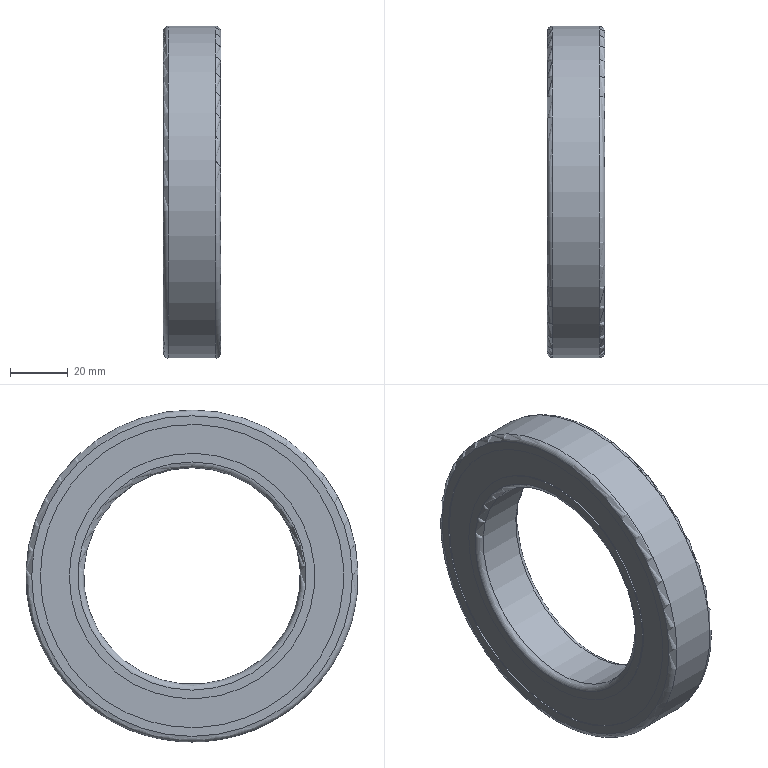Component | NX | BEARING_1 | 1 solid | 16 faces | box 20 x 115 x 115 mm | volume 115371 mm3 | plane 6 | cylinder 6 | torus 4 | commonest cylinder face diameters 105 x2 85 x2 115 x1 75 x1
STEP:
#1=CARTESIAN_POINT('',(0.,0.,0.));
#2=DIRECTION('',(0.,0.,1.));
#3=DIRECTION('',(1.,0.,0.));
#4=AXIS2_PLACEMENT_3D('',#1,#2,#3);
#5=CARTESIAN_POINT('',(1318.754,222.349,517.977));
#6=VERTEX_POINT('',#5);
#7=CARTESIAN_POINT('',(1318.754,222.349,478.477));
#8=DIRECTION('',(1.,0.,0.));
#9=DIRECTION('',(0.,0.,1.));
#10=AXIS2_PLACEMENT_3D('',#7,#8,#9);
#11=CIRCLE('',#10,39.5);
#12=CARTESIAN_POINT('',(1318.754,222.349,478.477));
#13=DIRECTION('',(1.,0.,0.));
#14=DIRECTION('',(0.,0.,1.));
#15=AXIS2_PLACEMENT_3D('',#12,#13,#14);
#16=PLANE('',#15);
#17=CARTESIAN_POINT('',(0.,0.));
#18=DIRECTION('',(1.,0.));
#19=AXIS2_PLACEMENT_2D('',#17,#18);
#20=CIRCLE('',#19,39.5);
#21=(GEOMETRIC_REPRESENTATION_CONTEXT(2)PARAMETRIC_REPRESENTATION_CONTEXT()REPRESENTATION_CONTEXT('',''));
#22=DEFINITIONAL_REPRESENTATION('',(#20),#21);
#23=PCURVE('',#16,#22);
#24=CARTESIAN_POINT('',(1320.754,222.349,478.477));
#25=DIRECTION('',(1.,0.,0.));
#26=DIRECTION('',(0.,0.,1.));
#27=AXIS2_PLACEMENT_3D('',#24,#25,#26);
#28=TOROIDAL_SURFACE('',#27,39.5,2.);
#29=CARTESIAN_POINT('',(0.,4.712));
#30=DIRECTION('',(1.,0.));
#31=VECTOR('',#30,1.);
#32=LINE('',#29,#31);
#33=(GEOMETRIC_REPRESENTATION_CONTEXT(2)PARAMETRIC_REPRESENTATION_CONTEXT()REPRESENTATION_CONTEXT('',''));
#34=DEFINITIONAL_REPRESENTATION('',(#32),#33);
#35=PCURVE('',#28,#34);
#36=SURFACE_CURVE('',#11,(#23,#35),.PCURVE_S1.);
#37=EDGE_CURVE('',#6,#6,#36,.T.);
#38=ORIENTED_EDGE('',*,*,#37,.T.);
#39=EDGE_LOOP('',(#38));
#40=FACE_BOUND('',#39,.T.);
#41=CARTESIAN_POINT('',(1318.754,264.849,478.477));
#42=VERTEX_POINT('',#41);
#43=CARTESIAN_POINT('',(1318.754,222.349,478.477));
#44=DIRECTION('',(-1.,0.,0.));
#45=DIRECTION('',(0.,1.,0.));
#46=AXIS2_PLACEMENT_3D('',#43,#44,#45);
#47=CIRCLE('',#46,42.5);
#48=CARTESIAN_POINT('',(0.,-42.5));
#49=CARTESIAN_POINT('',(-73.612,-42.5));
#50=CARTESIAN_POINT('',(-36.806,21.25));
#51=CARTESIAN_POINT('',(-0.,85.));
#52=CARTESIAN_POINT('',(36.806,21.25));
#53=CARTESIAN_POINT('',(73.612,-42.5));
#54=CARTESIAN_POINT('',(0.,-42.5));
#55=(BOUNDED_CURVE()B_SPLINE_CURVE(2,(#48,#49,#50,#51,#52,#53,#54),.UNSPECIFIED.,.T.,.F.)B_SPLINE_CURVE_WITH_KNOTS((1,2,2,2,2,1),(-2.094,0.,2.094,4.189,6.283,8.378),.UNSPECIFIED.)CURVE()GEOMETRIC_REPRESENTATION_ITEM()RATIONAL_B_SPLINE_CURVE((1.,0.5,1.,0.5,1.,0.5,1.))REPRESENTATION_ITEM(''));
#56=(GEOMETRIC_REPRESENTATION_CONTEXT(2)PARAMETRIC_REPRESENTATION_CONTEXT()REPRESENTATION_CONTEXT('',''));
#57=DEFINITIONAL_REPRESENTATION('',(#55),#56);
#58=PCURVE('',#16,#57);
#59=CARTESIAN_POINT('',(1319.254,222.349,478.477));
#60=DIRECTION('',(-1.,0.,0.));
#61=DIRECTION('',(0.,0.,-1.));
#62=AXIS2_PLACEMENT_3D('',#59,#60,#61);
#63=CYLINDRICAL_SURFACE('',#62,42.5);
#64=CARTESIAN_POINT('',(4.712,0.5));
#65=DIRECTION('',(1.,0.));
#66=VECTOR('',#65,1.);
#67=LINE('',#64,#66);
#68=(GEOMETRIC_REPRESENTATION_CONTEXT(2)PARAMETRIC_REPRESENTATION_CONTEXT()REPRESENTATION_CONTEXT('',''));
#69=DEFINITIONAL_REPRESENTATION('',(#67),#68);
#70=PCURVE('',#63,#69);
#71=SURFACE_CURVE('',#47,(#58,#70),.PCURVE_S1.);
#72=EDGE_CURVE('',#42,#42,#71,.T.);
#73=ORIENTED_EDGE('',*,*,#72,.T.);
#74=EDGE_LOOP('',(#73));
#75=FACE_BOUND('',#74,.T.);
#76=ADVANCED_FACE('',(#40,#75),#16,.F.);
#77=CARTESIAN_POINT('',(1320.754,222.349,535.977));
#78=VERTEX_POINT('',#77);
#79=CARTESIAN_POINT('',(1320.754,222.349,478.477));
#80=DIRECTION('',(1.,0.,0.));
#81=DIRECTION('',(0.,0.,1.));
#82=AXIS2_PLACEMENT_3D('',#79,#80,#81);
#83=CIRCLE('',#82,57.5);
#84=CARTESIAN_POINT('',(1328.754,222.349,478.477));
#85=DIRECTION('',(-1.,0.,0.));
#86=DIRECTION('',(0.,0.,-1.));
#87=AXIS2_PLACEMENT_3D('',#84,#85,#86);
#88=CYLINDRICAL_SURFACE('',#87,57.5);
#89=CARTESIAN_POINT('',(9.425,8.));
#90=DIRECTION('',(-1.,0.));
#91=VECTOR('',#90,1.);
#92=LINE('',#89,#91);
#93=(GEOMETRIC_REPRESENTATION_CONTEXT(2)PARAMETRIC_REPRESENTATION_CONTEXT()REPRESENTATION_CONTEXT('',''));
#94=DEFINITIONAL_REPRESENTATION('',(#92),#93);
#95=PCURVE('',#88,#94);
#96=CARTESIAN_POINT('',(1320.754,222.349,478.477));
#97=DIRECTION('',(1.,0.,0.));
#98=DIRECTION('',(0.,0.,1.));
#99=AXIS2_PLACEMENT_3D('',#96,#97,#98);
#100=TOROIDAL_SURFACE('',#99,55.5,2.);
#101=CARTESIAN_POINT('',(0.,6.283));
#102=DIRECTION('',(1.,0.));
#103=VECTOR('',#102,1.);
#104=LINE('',#101,#103);
#105=(GEOMETRIC_REPRESENTATION_CONTEXT(2)PARAMETRIC_REPRESENTATION_CONTEXT()REPRESENTATION_CONTEXT('',''));
#106=DEFINITIONAL_REPRESENTATION('',(#104),#105);
#107=PCURVE('',#100,#106);
#108=SURFACE_CURVE('',#83,(#95,#107),.PCURVE_S1.);
#109=EDGE_CURVE('',#78,#78,#108,.T.);
#110=ORIENTED_EDGE('',*,*,#109,.T.);
#111=CARTESIAN_POINT('',(1336.754,222.349,535.977));
#112=VERTEX_POINT('',#111);
#113=CARTESIAN_POINT('',(1336.754,222.349,535.977));
#114=CARTESIAN_POINT('',(1320.754,222.349,535.977));
#115=B_SPLINE_CURVE_WITH_KNOTS('',1,(#113,#114),.UNSPECIFIED.,.F.,.F.,(2,2),(-8.,8.),.PIECEWISE_BEZIER_KNOTS.);
#116=CARTESIAN_POINT('',(3.142,0.));
#117=DIRECTION('',(0.,1.));
#118=VECTOR('',#117,1.);
#119=LINE('',#116,#118);
#120=(GEOMETRIC_REPRESENTATION_CONTEXT(2)PARAMETRIC_REPRESENTATION_CONTEXT()REPRESENTATION_CONTEXT('',''));
#121=DEFINITIONAL_REPRESENTATION('',(#119),#120);
#122=PCURVE('',#88,#121);
#123=CARTESIAN_POINT('',(9.425,0.));
#124=DIRECTION('',(0.,1.));
#125=VECTOR('',#124,1.);
#126=LINE('',#123,#125);
#127=(GEOMETRIC_REPRESENTATION_CONTEXT(2)PARAMETRIC_REPRESENTATION_CONTEXT()REPRESENTATION_CONTEXT('',''));
#128=DEFINITIONAL_REPRESENTATION('',(#126),#127);
#129=PCURVE('',#88,#128);
#130=SEAM_CURVE('',#115,(#122,#129),.PCURVE_S1.);
#131=EDGE_CURVE('',#112,#78,#130,.T.);
#132=ORIENTED_EDGE('',*,*,#131,.F.);
#133=CARTESIAN_POINT('',(1336.754,222.349,478.477));
#134=DIRECTION('',(-1.,0.,0.));
#135=DIRECTION('',(0.,0.,1.));
#136=AXIS2_PLACEMENT_3D('',#133,#134,#135);
#137=CIRCLE('',#136,57.5);
#138=CARTESIAN_POINT('',(3.142,-8.));
#139=DIRECTION('',(1.,0.));
#140=VECTOR('',#139,1.);
#141=LINE('',#138,#140);
#142=(GEOMETRIC_REPRESENTATION_CONTEXT(2)PARAMETRIC_REPRESENTATION_CONTEXT()REPRESENTATION_CONTEXT('',''));
#143=DEFINITIONAL_REPRESENTATION('',(#141),#142);
#144=PCURVE('',#88,#143);
#145=CARTESIAN_POINT('',(1336.754,222.349,478.477));
#146=DIRECTION('',(-1.,0.,0.));
#147=DIRECTION('',(0.,0.,1.));
#148=AXIS2_PLACEMENT_3D('',#145,#146,#147);
#149=TOROIDAL_SURFACE('',#148,55.5,2.);
#150=CARTESIAN_POINT('',(0.,6.283));
#151=DIRECTION('',(1.,0.));
#152=VECTOR('',#151,1.);
#153=LINE('',#150,#152);
#154=(GEOMETRIC_REPRESENTATION_CONTEXT(2)PARAMETRIC_REPRESENTATION_CONTEXT()REPRESENTATION_CONTEXT('',''));
#155=DEFINITIONAL_REPRESENTATION('',(#153),#154);
#156=PCURVE('',#149,#155);
#157=SURFACE_CURVE('',#137,(#144,#156),.PCURVE_S1.);
#158=EDGE_CURVE('',#112,#112,#157,.T.);
#159=ORIENTED_EDGE('',*,*,#158,.T.);
#160=ORIENTED_EDGE('',*,*,#131,.T.);
#161=EDGE_LOOP('',(#110,#132,#159,#160));
#162=FACE_BOUND('',#161,.T.);
#163=ADVANCED_FACE('',(#162),#88,.T.);
#164=CARTESIAN_POINT('',(1320.754,222.349,515.977));
#165=VERTEX_POINT('',#164);
#166=CARTESIAN_POINT('',(1320.754,222.349,478.477));
#167=DIRECTION('',(-1.,0.,0.));
#168=DIRECTION('',(0.,0.,1.));
#169=AXIS2_PLACEMENT_3D('',#166,#167,#168);
#170=CIRCLE('',#169,37.5);
#171=CARTESIAN_POINT('',(1328.754,222.349,478.477));
#172=DIRECTION('',(-1.,0.,0.));
#173=DIRECTION('',(0.,0.,-1.));
#174=AXIS2_PLACEMENT_3D('',#171,#172,#173);
#175=CYLINDRICAL_SURFACE('',#174,37.5);
#176=CARTESIAN_POINT('',(3.142,8.));
#177=DIRECTION('',(1.,0.));
#178=VECTOR('',#177,1.);
#179=LINE('',#176,#178);
#180=(GEOMETRIC_REPRESENTATION_CONTEXT(2)PARAMETRIC_REPRESENTATION_CONTEXT()REPRESENTATION_CONTEXT('',''));
#181=DEFINITIONAL_REPRESENTATION('',(#179),#180);
#182=PCURVE('',#175,#181);
#183=CARTESIAN_POINT('',(6.283,3.142));
#184=DIRECTION('',(-1.,0.));
#185=VECTOR('',#184,1.);
#186=LINE('',#183,#185);
#187=(GEOMETRIC_REPRESENTATION_CONTEXT(2)PARAMETRIC_REPRESENTATION_CONTEXT()REPRESENTATION_CONTEXT('',''));
#188=DEFINITIONAL_REPRESENTATION('',(#186),#187);
#189=PCURVE('',#28,#188);
#190=SURFACE_CURVE('',#170,(#182,#189),.PCURVE_S1.);
#191=EDGE_CURVE('',#165,#165,#190,.T.);
#192=ORIENTED_EDGE('',*,*,#191,.F.);
#193=CARTESIAN_POINT('',(1336.754,222.349,515.977));
#194=VERTEX_POINT('',#193);
#195=CARTESIAN_POINT('',(1336.754,222.349,515.977));
#196=CARTESIAN_POINT('',(1320.754,222.349,515.977));
#197=B_SPLINE_CURVE_WITH_KNOTS('',1,(#195,#196),.UNSPECIFIED.,.F.,.F.,(2,2),(-8.,8.),.PIECEWISE_BEZIER_KNOTS.);
#198=CARTESIAN_POINT('',(3.142,0.));
#199=DIRECTION('',(0.,1.));
#200=VECTOR('',#199,1.);
#201=LINE('',#198,#200);
#202=(GEOMETRIC_REPRESENTATION_CONTEXT(2)PARAMETRIC_REPRESENTATION_CONTEXT()REPRESENTATION_CONTEXT('',''));
#203=DEFINITIONAL_REPRESENTATION('',(#201),#202);
#204=PCURVE('',#175,#203);
#205=CARTESIAN_POINT('',(9.425,0.));
#206=DIRECTION('',(0.,1.));
#207=VECTOR('',#206,1.);
#208=LINE('',#205,#207);
#209=(GEOMETRIC_REPRESENTATION_CONTEXT(2)PARAMETRIC_REPRESENTATION_CONTEXT()REPRESENTATION_CONTEXT('',''));
#210=DEFINITIONAL_REPRESENTATION('',(#208),#209);
#211=PCURVE('',#175,#210);
#212=SEAM_CURVE('',#197,(#204,#211),.PCURVE_S1.);
#213=EDGE_CURVE('',#194,#165,#212,.T.);
#214=ORIENTED_EDGE('',*,*,#213,.F.);
#215=CARTESIAN_POINT('',(1336.754,222.349,478.477));
#216=DIRECTION('',(1.,0.,0.));
#217=DIRECTION('',(0.,0.,1.));
#218=AXIS2_PLACEMENT_3D('',#215,#216,#217);
#219=CIRCLE('',#218,37.5);
#220=CARTESIAN_POINT('',(9.425,-8.));
#221=DIRECTION('',(-1.,0.));
#222=VECTOR('',#221,1.);
#223=LINE('',#220,#222);
#224=(GEOMETRIC_REPRESENTATION_CONTEXT(2)PARAMETRIC_REPRESENTATION_CONTEXT()REPRESENTATION_CONTEXT('',''));
#225=DEFINITIONAL_REPRESENTATION('',(#223),#224);
#226=PCURVE('',#175,#225);
#227=CARTESIAN_POINT('',(1336.754,222.349,478.477));
#228=DIRECTION('',(-1.,0.,0.));
#229=DIRECTION('',(0.,0.,1.));
#230=AXIS2_PLACEMENT_3D('',#227,#228,#229);
#231=TOROIDAL_SURFACE('',#230,39.5,2.);
#232=CARTESIAN_POINT('',(6.283,3.142));
#233=DIRECTION('',(-1.,0.));
#234=VECTOR('',#233,1.);
#235=LINE('',#232,#234);
#236=(GEOMETRIC_REPRESENTATION_CONTEXT(2)PARAMETRIC_REPRESENTATION_CONTEXT()REPRESENTATION_CONTEXT('',''));
#237=DEFINITIONAL_REPRESENTATION('',(#235),#236);
#238=PCURVE('',#231,#237);
#239=SURFACE_CURVE('',#219,(#226,#238),.PCURVE_S1.);
#240=EDGE_CURVE('',#194,#194,#239,.T.);
#241=ORIENTED_EDGE('',*,*,#240,.F.);
#242=ORIENTED_EDGE('',*,*,#213,.T.);
#243=EDGE_LOOP('',(#192,#214,#241,#242));
#244=FACE_BOUND('',#243,.F.);
#245=ADVANCED_FACE('',(#244),#175,.F.);
#246=CARTESIAN_POINT('',(1318.754,222.349,533.977));
#247=VERTEX_POINT('',#246);
#248=CARTESIAN_POINT('',(1318.754,222.349,478.477));
#249=DIRECTION('',(-1.,0.,0.));
#250=DIRECTION('',(0.,0.,1.));
#251=AXIS2_PLACEMENT_3D('',#248,#249,#250);
#252=CIRCLE('',#251,55.5);
#253=CARTESIAN_POINT('',(1318.754,222.349,478.477));
#254=DIRECTION('',(1.,0.,0.));
#255=DIRECTION('',(0.,0.,1.));
#256=AXIS2_PLACEMENT_3D('',#253,#254,#255);
#257=PLANE('',#256);
#258=CARTESIAN_POINT('',(55.5,0.));
#259=CARTESIAN_POINT('',(55.5,-96.129));
#260=CARTESIAN_POINT('',(-27.75,-48.064));
#261=CARTESIAN_POINT('',(-111.,-0.));
#262=CARTESIAN_POINT('',(-27.75,48.064));
#263=CARTESIAN_POINT('',(55.5,96.129));
#264=CARTESIAN_POINT('',(55.5,0.));
#265=(BOUNDED_CURVE()B_SPLINE_CURVE(2,(#258,#259,#260,#261,#262,#263,#264),.UNSPECIFIED.,.T.,.F.)B_SPLINE_CURVE_WITH_KNOTS((1,2,2,2,2,1),(-2.094,0.,2.094,4.189,6.283,8.378),.UNSPECIFIED.)CURVE()GEOMETRIC_REPRESENTATION_ITEM()RATIONAL_B_SPLINE_CURVE((1.,0.5,1.,0.5,1.,0.5,1.))REPRESENTATION_ITEM(''));
#266=(GEOMETRIC_REPRESENTATION_CONTEXT(2)PARAMETRIC_REPRESENTATION_CONTEXT()REPRESENTATION_CONTEXT('',''));
#267=DEFINITIONAL_REPRESENTATION('',(#265),#266);
#268=PCURVE('',#257,#267);
#269=CARTESIAN_POINT('',(6.283,4.712));
#270=DIRECTION('',(-1.,0.));
#271=VECTOR('',#270,1.);
#272=LINE('',#269,#271);
#273=(GEOMETRIC_REPRESENTATION_CONTEXT(2)PARAMETRIC_REPRESENTATION_CONTEXT()REPRESENTATION_CONTEXT('',''));
#274=DEFINITIONAL_REPRESENTATION('',(#272),#273);
#275=PCURVE('',#100,#274);
#276=SURFACE_CURVE('',#252,(#268,#275),.PCURVE_S1.);
#277=EDGE_CURVE('',#247,#247,#276,.T.);
#278=ORIENTED_EDGE('',*,*,#277,.T.);
#279=EDGE_LOOP('',(#278));
#280=FACE_BOUND('',#279,.T.);
#281=CARTESIAN_POINT('',(1318.754,274.849,478.477));
#282=VERTEX_POINT('',#281);
#283=CARTESIAN_POINT('',(1318.754,222.349,478.477));
#284=DIRECTION('',(-1.,0.,0.));
#285=DIRECTION('',(0.,1.,0.));
#286=AXIS2_PLACEMENT_3D('',#283,#284,#285);
#287=CIRCLE('',#286,52.5);
#288=CARTESIAN_POINT('',(0.,-52.5));
#289=CARTESIAN_POINT('',(-90.933,-52.5));
#290=CARTESIAN_POINT('',(-45.466,26.25));
#291=CARTESIAN_POINT('',(-0.,105.));
#292=CARTESIAN_POINT('',(45.466,26.25));
#293=CARTESIAN_POINT('',(90.933,-52.5));
#294=CARTESIAN_POINT('',(0.,-52.5));
#295=(BOUNDED_CURVE()B_SPLINE_CURVE(2,(#288,#289,#290,#291,#292,#293,#294),.UNSPECIFIED.,.T.,.F.)B_SPLINE_CURVE_WITH_KNOTS((1,2,2,2,2,1),(-2.094,0.,2.094,4.189,6.283,8.378),.UNSPECIFIED.)CURVE()GEOMETRIC_REPRESENTATION_ITEM()RATIONAL_B_SPLINE_CURVE((1.,0.5,1.,0.5,1.,0.5,1.))REPRESENTATION_ITEM(''));
#296=(GEOMETRIC_REPRESENTATION_CONTEXT(2)PARAMETRIC_REPRESENTATION_CONTEXT()REPRESENTATION_CONTEXT('',''));
#297=DEFINITIONAL_REPRESENTATION('',(#295),#296);
#298=PCURVE('',#257,#297);
#299=CARTESIAN_POINT('',(1319.254,222.349,478.477));
#300=DIRECTION('',(-1.,0.,0.));
#301=DIRECTION('',(0.,0.,-1.));
#302=AXIS2_PLACEMENT_3D('',#299,#300,#301);
#303=CYLINDRICAL_SURFACE('',#302,52.5);
#304=CARTESIAN_POINT('',(4.712,0.5));
#305=DIRECTION('',(1.,0.));
#306=VECTOR('',#305,1.);
#307=LINE('',#304,#306);
#308=(GEOMETRIC_REPRESENTATION_CONTEXT(2)PARAMETRIC_REPRESENTATION_CONTEXT()REPRESENTATION_CONTEXT('',''));
#309=DEFINITIONAL_REPRESENTATION('',(#307),#308);
#310=PCURVE('',#303,#309);
#311=SURFACE_CURVE('',#287,(#298,#310),.PCURVE_S1.);
#312=EDGE_CURVE('',#282,#282,#311,.T.);
#313=ORIENTED_EDGE('',*,*,#312,.F.);
#314=EDGE_LOOP('',(#313));
#315=FACE_BOUND('',#314,.T.);
#316=ADVANCED_FACE('',(#280,#315),#257,.F.);
#317=CARTESIAN_POINT('',(1319.254,274.849,478.477));
#318=VERTEX_POINT('',#317);
#319=CARTESIAN_POINT('',(1319.254,222.349,478.477));
#320=DIRECTION('',(1.,0.,0.));
#321=DIRECTION('',(0.,1.,0.));
#322=AXIS2_PLACEMENT_3D('',#319,#320,#321);
#323=CIRCLE('',#322,52.5);
#324=CARTESIAN_POINT('',(10.996,0.));
#325=DIRECTION('',(-1.,0.));
#326=VECTOR('',#325,1.);
#327=LINE('',#324,#326);
#328=(GEOMETRIC_REPRESENTATION_CONTEXT(2)PARAMETRIC_REPRESENTATION_CONTEXT()REPRESENTATION_CONTEXT('',''));
#329=DEFINITIONAL_REPRESENTATION('',(#327),#328);
#330=PCURVE('',#303,#329);
#331=CARTESIAN_POINT('',(1319.254,222.349,478.477));
#332=DIRECTION('',(-1.,0.,0.));
#333=DIRECTION('',(0.,0.,-1.));
#334=AXIS2_PLACEMENT_3D('',#331,#332,#333);
#335=PLANE('',#334);
#336=CARTESIAN_POINT('',(0.,-52.5));
#337=CARTESIAN_POINT('',(-90.933,-52.5));
#338=CARTESIAN_POINT('',(-45.466,26.25));
#339=CARTESIAN_POINT('',(-0.,105.));
#340=CARTESIAN_POINT('',(45.466,26.25));
#341=CARTESIAN_POINT('',(90.933,-52.5));
#342=CARTESIAN_POINT('',(0.,-52.5));
#343=(BOUNDED_CURVE()B_SPLINE_CURVE(2,(#336,#337,#338,#339,#340,#341,#342),.UNSPECIFIED.,.T.,.F.)B_SPLINE_CURVE_WITH_KNOTS((1,2,2,2,2,1),(-2.094,0.,2.094,4.189,6.283,8.378),.UNSPECIFIED.)CURVE()GEOMETRIC_REPRESENTATION_ITEM()RATIONAL_B_SPLINE_CURVE((1.,0.5,1.,0.5,1.,0.5,1.))REPRESENTATION_ITEM(''));
#344=(GEOMETRIC_REPRESENTATION_CONTEXT(2)PARAMETRIC_REPRESENTATION_CONTEXT()REPRESENTATION_CONTEXT('',''));
#345=DEFINITIONAL_REPRESENTATION('',(#343),#344);
#346=PCURVE('',#335,#345);
#347=SURFACE_CURVE('',#323,(#330,#346),.PCURVE_S1.);
#348=EDGE_CURVE('',#318,#318,#347,.T.);
#349=ORIENTED_EDGE('',*,*,#348,.F.);
#350=CARTESIAN_POINT('',(1319.254,274.849,478.477));
#351=CARTESIAN_POINT('',(1318.754,274.849,478.477));
#352=B_SPLINE_CURVE_WITH_KNOTS('',1,(#350,#351),.UNSPECIFIED.,.F.,.F.,(2,2),(0.,0.5),.PIECEWISE_BEZIER_KNOTS.);
#353=CARTESIAN_POINT('',(10.996,0.));
#354=DIRECTION('',(0.,1.));
#355=VECTOR('',#354,1.);
#356=LINE('',#353,#355);
#357=(GEOMETRIC_REPRESENTATION_CONTEXT(2)PARAMETRIC_REPRESENTATION_CONTEXT()REPRESENTATION_CONTEXT('',''));
#358=DEFINITIONAL_REPRESENTATION('',(#356),#357);
#359=PCURVE('',#303,#358);
#360=CARTESIAN_POINT('',(4.712,0.));
#361=DIRECTION('',(0.,1.));
#362=VECTOR('',#361,1.);
#363=LINE('',#360,#362);
#364=(GEOMETRIC_REPRESENTATION_CONTEXT(2)PARAMETRIC_REPRESENTATION_CONTEXT()REPRESENTATION_CONTEXT('',''));
#365=DEFINITIONAL_REPRESENTATION('',(#363),#364);
#366=PCURVE('',#303,#365);
#367=SEAM_CURVE('',#352,(#359,#366),.PCURVE_S1.);
#368=EDGE_CURVE('',#318,#282,#367,.T.);
#369=ORIENTED_EDGE('',*,*,#368,.T.);
#370=ORIENTED_EDGE('',*,*,#312,.F.);
#371=ORIENTED_EDGE('',*,*,#368,.F.);
#372=EDGE_LOOP('',(#349,#369,#370,#371));
#373=FACE_BOUND('',#372,.F.);
#374=ADVANCED_FACE('',(#373),#303,.F.);
#375=CARTESIAN_POINT('',(1319.254,264.849,478.477));
#376=VERTEX_POINT('',#375);
#377=CARTESIAN_POINT('',(1319.254,222.349,478.477));
#378=DIRECTION('',(1.,0.,0.));
#379=DIRECTION('',(0.,1.,0.));
#380=AXIS2_PLACEMENT_3D('',#377,#378,#379);
#381=CIRCLE('',#380,42.5);
#382=CARTESIAN_POINT('',(10.996,0.));
#383=DIRECTION('',(-1.,0.));
#384=VECTOR('',#383,1.);
#385=LINE('',#382,#384);
#386=(GEOMETRIC_REPRESENTATION_CONTEXT(2)PARAMETRIC_REPRESENTATION_CONTEXT()REPRESENTATION_CONTEXT('',''));
#387=DEFINITIONAL_REPRESENTATION('',(#385),#386);
#388=PCURVE('',#63,#387);
#389=CARTESIAN_POINT('',(0.,-42.5));
#390=CARTESIAN_POINT('',(-73.612,-42.5));
#391=CARTESIAN_POINT('',(-36.806,21.25));
#392=CARTESIAN_POINT('',(-0.,85.));
#393=CARTESIAN_POINT('',(36.806,21.25));
#394=CARTESIAN_POINT('',(73.612,-42.5));
#395=CARTESIAN_POINT('',(0.,-42.5));
#396=(BOUNDED_CURVE()B_SPLINE_CURVE(2,(#389,#390,#391,#392,#393,#394,#395),.UNSPECIFIED.,.T.,.F.)B_SPLINE_CURVE_WITH_KNOTS((1,2,2,2,2,1),(-2.094,0.,2.094,4.189,6.283,8.378),.UNSPECIFIED.)CURVE()GEOMETRIC_REPRESENTATION_ITEM()RATIONAL_B_SPLINE_CURVE((1.,0.5,1.,0.5,1.,0.5,1.))REPRESENTATION_ITEM(''));
#397=(GEOMETRIC_REPRESENTATION_CONTEXT(2)PARAMETRIC_REPRESENTATION_CONTEXT()REPRESENTATION_CONTEXT('',''));
#398=DEFINITIONAL_REPRESENTATION('',(#396),#397);
#399=PCURVE('',#335,#398);
#400=SURFACE_CURVE('',#381,(#388,#399),.PCURVE_S1.);
#401=EDGE_CURVE('',#376,#376,#400,.T.);
#402=ORIENTED_EDGE('',*,*,#401,.F.);
#403=CARTESIAN_POINT('',(1319.254,264.849,478.477));
#404=CARTESIAN_POINT('',(1318.754,264.849,478.477));
#405=B_SPLINE_CURVE_WITH_KNOTS('',1,(#403,#404),.UNSPECIFIED.,.F.,.F.,(2,2),(0.,0.5),.PIECEWISE_BEZIER_KNOTS.);
#406=CARTESIAN_POINT('',(10.996,0.));
#407=DIRECTION('',(0.,1.));
#408=VECTOR('',#407,1.);
#409=LINE('',#406,#408);
#410=(GEOMETRIC_REPRESENTATION_CONTEXT(2)PARAMETRIC_REPRESENTATION_CONTEXT()REPRESENTATION_CONTEXT('',''));
#411=DEFINITIONAL_REPRESENTATION('',(#409),#410);
#412=PCURVE('',#63,#411);
#413=CARTESIAN_POINT('',(4.712,0.));
#414=DIRECTION('',(0.,1.));
#415=VECTOR('',#414,1.);
#416=LINE('',#413,#415);
#417=(GEOMETRIC_REPRESENTATION_CONTEXT(2)PARAMETRIC_REPRESENTATION_CONTEXT()REPRESENTATION_CONTEXT('',''));
#418=DEFINITIONAL_REPRESENTATION('',(#416),#417);
#419=PCURVE('',#63,#418);
#420=SEAM_CURVE('',#405,(#412,#419),.PCURVE_S1.);
#421=EDGE_CURVE('',#376,#42,#420,.T.);
#422=ORIENTED_EDGE('',*,*,#421,.T.);
#423=ORIENTED_EDGE('',*,*,#72,.F.);
#424=ORIENTED_EDGE('',*,*,#421,.F.);
#425=EDGE_LOOP('',(#402,#422,#423,#424));
#426=FACE_BOUND('',#425,.T.);
#427=ADVANCED_FACE('',(#426),#63,.T.);
#428=ORIENTED_EDGE('',*,*,#348,.F.);
#429=EDGE_LOOP('',(#428));
#430=FACE_BOUND('',#429,.T.);
#431=ORIENTED_EDGE('',*,*,#401,.T.);
#432=EDGE_LOOP('',(#431));
#433=FACE_BOUND('',#432,.T.);
#434=ADVANCED_FACE('',(#430,#433),#335,.T.);
#435=ORIENTED_EDGE('',*,*,#37,.F.);
#436=CARTESIAN_POINT('',(1320.754,222.349,515.977));
#437=CARTESIAN_POINT('',(1320.219,222.349,515.977));
#438=CARTESIAN_POINT('',(1319.699,222.349,516.147));
#439=CARTESIAN_POINT('',(1319.25,222.349,516.473));
#440=CARTESIAN_POINT('',(1318.924,222.349,516.921));
#441=CARTESIAN_POINT('',(1318.754,222.349,517.442));
#442=CARTESIAN_POINT('',(1318.754,222.349,517.977));
#443=(BOUNDED_CURVE()B_SPLINE_CURVE(6,(#436,#437,#438,#439,#440,#441,#442),.UNSPECIFIED.,.F.,.F.)B_SPLINE_CURVE_WITH_KNOTS((7,7),(3.142,4.712),.PIECEWISE_BEZIER_KNOTS.)CURVE()GEOMETRIC_REPRESENTATION_ITEM()RATIONAL_B_SPLINE_CURVE((1.031,1.01,0.9979,0.994,0.9979,1.01,1.031))REPRESENTATION_ITEM(''));
#444=CARTESIAN_POINT('',(0.,0.));
#445=DIRECTION('',(0.,1.));
#446=VECTOR('',#445,1.);
#447=LINE('',#444,#446);
#448=(GEOMETRIC_REPRESENTATION_CONTEXT(2)PARAMETRIC_REPRESENTATION_CONTEXT()REPRESENTATION_CONTEXT('',''));
#449=DEFINITIONAL_REPRESENTATION('',(#447),#448);
#450=PCURVE('',#28,#449);
#451=CARTESIAN_POINT('',(6.283,0.));
#452=DIRECTION('',(0.,1.));
#453=VECTOR('',#452,1.);
#454=LINE('',#451,#453);
#455=(GEOMETRIC_REPRESENTATION_CONTEXT(2)PARAMETRIC_REPRESENTATION_CONTEXT()REPRESENTATION_CONTEXT('',''));
#456=DEFINITIONAL_REPRESENTATION('',(#454),#455);
#457=PCURVE('',#28,#456);
#458=SEAM_CURVE('',#443,(#450,#457),.PCURVE_S1.);
#459=EDGE_CURVE('',#165,#6,#458,.T.);
#460=ORIENTED_EDGE('',*,*,#459,.F.);
#461=ORIENTED_EDGE('',*,*,#191,.F.);
#462=ORIENTED_EDGE('',*,*,#459,.T.);
#463=EDGE_LOOP('',(#435,#460,#461,#462));
#464=FACE_BOUND('',#463,.T.);
#465=ADVANCED_FACE('',(#464),#28,.T.);
#466=ORIENTED_EDGE('',*,*,#109,.F.);
#467=CARTESIAN_POINT('',(1318.754,222.349,533.977));
#468=CARTESIAN_POINT('',(1318.754,222.349,534.512));
#469=CARTESIAN_POINT('',(1318.924,222.349,535.032));
#470=CARTESIAN_POINT('',(1319.25,222.349,535.481));
#471=CARTESIAN_POINT('',(1319.699,222.349,535.807));
#472=CARTESIAN_POINT('',(1320.219,222.349,535.977));
#473=CARTESIAN_POINT('',(1320.754,222.349,535.977));
#474=(BOUNDED_CURVE()B_SPLINE_CURVE(6,(#467,#468,#469,#470,#471,#472,#473),.UNSPECIFIED.,.F.,.F.)B_SPLINE_CURVE_WITH_KNOTS((7,7),(-1.571,0.),.PIECEWISE_BEZIER_KNOTS.)CURVE()GEOMETRIC_REPRESENTATION_ITEM()RATIONAL_B_SPLINE_CURVE((1.031,1.01,0.9979,0.994,0.9979,1.01,1.031))REPRESENTATION_ITEM(''));
#475=CARTESIAN_POINT('',(0.,6.283));
#476=DIRECTION('',(0.,1.));
#477=VECTOR('',#476,1.);
#478=LINE('',#475,#477);
#479=(GEOMETRIC_REPRESENTATION_CONTEXT(2)PARAMETRIC_REPRESENTATION_CONTEXT()REPRESENTATION_CONTEXT('',''));
#480=DEFINITIONAL_REPRESENTATION('',(#478),#479);
#481=PCURVE('',#100,#480);
#482=CARTESIAN_POINT('',(6.283,6.283));
#483=DIRECTION('',(0.,1.));
#484=VECTOR('',#483,1.);
#485=LINE('',#482,#484);
#486=(GEOMETRIC_REPRESENTATION_CONTEXT(2)PARAMETRIC_REPRESENTATION_CONTEXT()REPRESENTATION_CONTEXT('',''));
#487=DEFINITIONAL_REPRESENTATION('',(#485),#486);
#488=PCURVE('',#100,#487);
#489=SEAM_CURVE('',#474,(#481,#488),.PCURVE_S1.);
#490=EDGE_CURVE('',#247,#78,#489,.T.);
#491=ORIENTED_EDGE('',*,*,#490,.F.);
#492=ORIENTED_EDGE('',*,*,#277,.F.);
#493=ORIENTED_EDGE('',*,*,#490,.T.);
#494=EDGE_LOOP('',(#466,#491,#492,#493));
#495=FACE_BOUND('',#494,.T.);
#496=ADVANCED_FACE('',(#495),#100,.T.);
#497=CARTESIAN_POINT('',(1338.754,222.349,517.977));
#498=VERTEX_POINT('',#497);
#499=CARTESIAN_POINT('',(1338.754,222.349,478.477));
#500=DIRECTION('',(-1.,0.,0.));
#501=DIRECTION('',(0.,0.,1.));
#502=AXIS2_PLACEMENT_3D('',#499,#500,#501);
#503=CIRCLE('',#502,39.5);
#504=CARTESIAN_POINT('',(1338.754,222.349,478.477));
#505=DIRECTION('',(-1.,0.,0.));
#506=DIRECTION('',(0.,0.,1.));
#507=AXIS2_PLACEMENT_3D('',#504,#505,#506);
#508=PLANE('',#507);
#509=CARTESIAN_POINT('',(0.,0.));
#510=DIRECTION('',(1.,0.));
#511=AXIS2_PLACEMENT_2D('',#509,#510);
#512=CIRCLE('',#511,39.5);
#513=(GEOMETRIC_REPRESENTATION_CONTEXT(2)PARAMETRIC_REPRESENTATION_CONTEXT()REPRESENTATION_CONTEXT('',''));
#514=DEFINITIONAL_REPRESENTATION('',(#512),#513);
#515=PCURVE('',#508,#514);
#516=CARTESIAN_POINT('',(0.,4.712));
#517=DIRECTION('',(1.,0.));
#518=VECTOR('',#517,1.);
#519=LINE('',#516,#518);
#520=(GEOMETRIC_REPRESENTATION_CONTEXT(2)PARAMETRIC_REPRESENTATION_CONTEXT()REPRESENTATION_CONTEXT('',''));
#521=DEFINITIONAL_REPRESENTATION('',(#519),#520);
#522=PCURVE('',#231,#521);
#523=SURFACE_CURVE('',#503,(#515,#522),.PCURVE_S1.);
#524=EDGE_CURVE('',#498,#498,#523,.T.);
#525=ORIENTED_EDGE('',*,*,#524,.T.);
#526=EDGE_LOOP('',(#525));
#527=FACE_BOUND('',#526,.T.);
#528=CARTESIAN_POINT('',(1338.754,264.849,478.477));
#529=VERTEX_POINT('',#528);
#530=CARTESIAN_POINT('',(1338.754,222.349,478.477));
#531=DIRECTION('',(1.,0.,0.));
#532=DIRECTION('',(0.,1.,0.));
#533=AXIS2_PLACEMENT_3D('',#530,#531,#532);
#534=CIRCLE('',#533,42.5);
#535=CARTESIAN_POINT('',(0.,42.5));
#536=CARTESIAN_POINT('',(73.612,42.5));
#537=CARTESIAN_POINT('',(36.806,-21.25));
#538=CARTESIAN_POINT('',(0.,-85.));
#539=CARTESIAN_POINT('',(-36.806,-21.25));
#540=CARTESIAN_POINT('',(-73.612,42.5));
#541=CARTESIAN_POINT('',(0.,42.5));
#542=(BOUNDED_CURVE()B_SPLINE_CURVE(2,(#535,#536,#537,#538,#539,#540,#541),.UNSPECIFIED.,.T.,.F.)B_SPLINE_CURVE_WITH_KNOTS((1,2,2,2,2,1),(-2.094,0.,2.094,4.189,6.283,8.378),.UNSPECIFIED.)CURVE()GEOMETRIC_REPRESENTATION_ITEM()RATIONAL_B_SPLINE_CURVE((1.,0.5,1.,0.5,1.,0.5,1.))REPRESENTATION_ITEM(''));
#543=(GEOMETRIC_REPRESENTATION_CONTEXT(2)PARAMETRIC_REPRESENTATION_CONTEXT()REPRESENTATION_CONTEXT('',''));
#544=DEFINITIONAL_REPRESENTATION('',(#542),#543);
#545=PCURVE('',#508,#544);
#546=CARTESIAN_POINT('',(1338.254,222.349,478.477));
#547=DIRECTION('',(1.,0.,0.));
#548=DIRECTION('',(0.,0.,-1.));
#549=AXIS2_PLACEMENT_3D('',#546,#547,#548);
#550=CYLINDRICAL_SURFACE('',#549,42.5);
#551=CARTESIAN_POINT('',(1.571,0.5));
#552=DIRECTION('',(1.,0.));
#553=VECTOR('',#552,1.);
#554=LINE('',#551,#553);
#555=(GEOMETRIC_REPRESENTATION_CONTEXT(2)PARAMETRIC_REPRESENTATION_CONTEXT()REPRESENTATION_CONTEXT('',''));
#556=DEFINITIONAL_REPRESENTATION('',(#554),#555);
#557=PCURVE('',#550,#556);
#558=SURFACE_CURVE('',#534,(#545,#557),.PCURVE_S1.);
#559=EDGE_CURVE('',#529,#529,#558,.T.);
#560=ORIENTED_EDGE('',*,*,#559,.T.);
#561=EDGE_LOOP('',(#560));
#562=FACE_BOUND('',#561,.T.);
#563=ADVANCED_FACE('',(#527,#562),#508,.F.);
#564=CARTESIAN_POINT('',(1338.754,222.349,533.977));
#565=VERTEX_POINT('',#564);
#566=CARTESIAN_POINT('',(1338.754,222.349,478.477));
#567=DIRECTION('',(1.,0.,0.));
#568=DIRECTION('',(0.,0.,1.));
#569=AXIS2_PLACEMENT_3D('',#566,#567,#568);
#570=CIRCLE('',#569,55.5);
#571=CARTESIAN_POINT('',(1338.754,222.349,478.477));
#572=DIRECTION('',(-1.,0.,0.));
#573=DIRECTION('',(0.,0.,1.));
#574=AXIS2_PLACEMENT_3D('',#571,#572,#573);
#575=PLANE('',#574);
#576=CARTESIAN_POINT('',(55.5,0.));
#577=CARTESIAN_POINT('',(55.5,-96.129));
#578=CARTESIAN_POINT('',(-27.75,-48.064));
#579=CARTESIAN_POINT('',(-111.,-0.));
#580=CARTESIAN_POINT('',(-27.75,48.064));
#581=CARTESIAN_POINT('',(55.5,96.129));
#582=CARTESIAN_POINT('',(55.5,0.));
#583=(BOUNDED_CURVE()B_SPLINE_CURVE(2,(#576,#577,#578,#579,#580,#581,#582),.UNSPECIFIED.,.T.,.F.)B_SPLINE_CURVE_WITH_KNOTS((1,2,2,2,2,1),(-2.094,0.,2.094,4.189,6.283,8.378),.UNSPECIFIED.)CURVE()GEOMETRIC_REPRESENTATION_ITEM()RATIONAL_B_SPLINE_CURVE((1.,0.5,1.,0.5,1.,0.5,1.))REPRESENTATION_ITEM(''));
#584=(GEOMETRIC_REPRESENTATION_CONTEXT(2)PARAMETRIC_REPRESENTATION_CONTEXT()REPRESENTATION_CONTEXT('',''));
#585=DEFINITIONAL_REPRESENTATION('',(#583),#584);
#586=PCURVE('',#575,#585);
#587=CARTESIAN_POINT('',(6.283,4.712));
#588=DIRECTION('',(-1.,0.));
#589=VECTOR('',#588,1.);
#590=LINE('',#587,#589);
#591=(GEOMETRIC_REPRESENTATION_CONTEXT(2)PARAMETRIC_REPRESENTATION_CONTEXT()REPRESENTATION_CONTEXT('',''));
#592=DEFINITIONAL_REPRESENTATION('',(#590),#591);
#593=PCURVE('',#149,#592);
#594=SURFACE_CURVE('',#570,(#586,#593),.PCURVE_S1.);
#595=EDGE_CURVE('',#565,#565,#594,.T.);
#596=ORIENTED_EDGE('',*,*,#595,.T.);
#597=EDGE_LOOP('',(#596));
#598=FACE_BOUND('',#597,.T.);
#599=CARTESIAN_POINT('',(1338.754,274.849,478.477));
#600=VERTEX_POINT('',#599);
#601=CARTESIAN_POINT('',(1338.754,222.349,478.477));
#602=DIRECTION('',(1.,0.,0.));
#603=DIRECTION('',(0.,1.,0.));
#604=AXIS2_PLACEMENT_3D('',#601,#602,#603);
#605=CIRCLE('',#604,52.5);
#606=CARTESIAN_POINT('',(0.,52.5));
#607=CARTESIAN_POINT('',(90.933,52.5));
#608=CARTESIAN_POINT('',(45.466,-26.25));
#609=CARTESIAN_POINT('',(0.,-105.));
#610=CARTESIAN_POINT('',(-45.466,-26.25));
#611=CARTESIAN_POINT('',(-90.933,52.5));
#612=CARTESIAN_POINT('',(0.,52.5));
#613=(BOUNDED_CURVE()B_SPLINE_CURVE(2,(#606,#607,#608,#609,#610,#611,#612),.UNSPECIFIED.,.T.,.F.)B_SPLINE_CURVE_WITH_KNOTS((1,2,2,2,2,1),(-2.094,0.,2.094,4.189,6.283,8.378),.UNSPECIFIED.)CURVE()GEOMETRIC_REPRESENTATION_ITEM()RATIONAL_B_SPLINE_CURVE((1.,0.5,1.,0.5,1.,0.5,1.))REPRESENTATION_ITEM(''));
#614=(GEOMETRIC_REPRESENTATION_CONTEXT(2)PARAMETRIC_REPRESENTATION_CONTEXT()REPRESENTATION_CONTEXT('',''));
#615=DEFINITIONAL_REPRESENTATION('',(#613),#614);
#616=PCURVE('',#575,#615);
#617=CARTESIAN_POINT('',(1338.254,222.349,478.477));
#618=DIRECTION('',(1.,0.,0.));
#619=DIRECTION('',(0.,0.,-1.));
#620=AXIS2_PLACEMENT_3D('',#617,#618,#619);
#621=CYLINDRICAL_SURFACE('',#620,52.5);
#622=CARTESIAN_POINT('',(1.571,0.5));
#623=DIRECTION('',(1.,0.));
#624=VECTOR('',#623,1.);
#625=LINE('',#622,#624);
#626=(GEOMETRIC_REPRESENTATION_CONTEXT(2)PARAMETRIC_REPRESENTATION_CONTEXT()REPRESENTATION_CONTEXT('',''));
#627=DEFINITIONAL_REPRESENTATION('',(#625),#626);
#628=PCURVE('',#621,#627);
#629=SURFACE_CURVE('',#605,(#616,#628),.PCURVE_S1.);
#630=EDGE_CURVE('',#600,#600,#629,.T.);
#631=ORIENTED_EDGE('',*,*,#630,.F.);
#632=EDGE_LOOP('',(#631));
#633=FACE_BOUND('',#632,.T.);
#634=ADVANCED_FACE('',(#598,#633),#575,.F.);
#635=CARTESIAN_POINT('',(1338.254,274.849,478.477));
#636=VERTEX_POINT('',#635);
#637=CARTESIAN_POINT('',(1338.254,222.349,478.477));
#638=DIRECTION('',(-1.,0.,0.));
#639=DIRECTION('',(0.,1.,0.));
#640=AXIS2_PLACEMENT_3D('',#637,#638,#639);
#641=CIRCLE('',#640,52.5);
#642=CARTESIAN_POINT('',(7.854,0.));
#643=DIRECTION('',(-1.,0.));
#644=VECTOR('',#643,1.);
#645=LINE('',#642,#644);
#646=(GEOMETRIC_REPRESENTATION_CONTEXT(2)PARAMETRIC_REPRESENTATION_CONTEXT()REPRESENTATION_CONTEXT('',''));
#647=DEFINITIONAL_REPRESENTATION('',(#645),#646);
#648=PCURVE('',#621,#647);
#649=CARTESIAN_POINT('',(1338.254,222.349,478.477));
#650=DIRECTION('',(1.,0.,0.));
#651=DIRECTION('',(0.,0.,-1.));
#652=AXIS2_PLACEMENT_3D('',#649,#650,#651);
#653=PLANE('',#652);
#654=CARTESIAN_POINT('',(0.,52.5));
#655=CARTESIAN_POINT('',(90.933,52.5));
#656=CARTESIAN_POINT('',(45.466,-26.25));
#657=CARTESIAN_POINT('',(0.,-105.));
#658=CARTESIAN_POINT('',(-45.466,-26.25));
#659=CARTESIAN_POINT('',(-90.933,52.5));
#660=CARTESIAN_POINT('',(0.,52.5));
#661=(BOUNDED_CURVE()B_SPLINE_CURVE(2,(#654,#655,#656,#657,#658,#659,#660),.UNSPECIFIED.,.T.,.F.)B_SPLINE_CURVE_WITH_KNOTS((1,2,2,2,2,1),(-2.094,0.,2.094,4.189,6.283,8.378),.UNSPECIFIED.)CURVE()GEOMETRIC_REPRESENTATION_ITEM()RATIONAL_B_SPLINE_CURVE((1.,0.5,1.,0.5,1.,0.5,1.))REPRESENTATION_ITEM(''));
#662=(GEOMETRIC_REPRESENTATION_CONTEXT(2)PARAMETRIC_REPRESENTATION_CONTEXT()REPRESENTATION_CONTEXT('',''));
#663=DEFINITIONAL_REPRESENTATION('',(#661),#662);
#664=PCURVE('',#653,#663);
#665=SURFACE_CURVE('',#641,(#648,#664),.PCURVE_S1.);
#666=EDGE_CURVE('',#636,#636,#665,.T.);
#667=ORIENTED_EDGE('',*,*,#666,.F.);
#668=CARTESIAN_POINT('',(1338.254,274.849,478.477));
#669=CARTESIAN_POINT('',(1338.754,274.849,478.477));
#670=B_SPLINE_CURVE_WITH_KNOTS('',1,(#668,#669),.UNSPECIFIED.,.F.,.F.,(2,2),(0.,0.5),.PIECEWISE_BEZIER_KNOTS.);
#671=CARTESIAN_POINT('',(7.854,0.));
#672=DIRECTION('',(0.,1.));
#673=VECTOR('',#672,1.);
#674=LINE('',#671,#673);
#675=(GEOMETRIC_REPRESENTATION_CONTEXT(2)PARAMETRIC_REPRESENTATION_CONTEXT()REPRESENTATION_CONTEXT('',''));
#676=DEFINITIONAL_REPRESENTATION('',(#674),#675);
#677=PCURVE('',#621,#676);
#678=CARTESIAN_POINT('',(1.571,0.));
#679=DIRECTION('',(0.,1.));
#680=VECTOR('',#679,1.);
#681=LINE('',#678,#680);
#682=(GEOMETRIC_REPRESENTATION_CONTEXT(2)PARAMETRIC_REPRESENTATION_CONTEXT()REPRESENTATION_CONTEXT('',''));
#683=DEFINITIONAL_REPRESENTATION('',(#681),#682);
#684=PCURVE('',#621,#683);
#685=SEAM_CURVE('',#670,(#677,#684),.PCURVE_S1.);
#686=EDGE_CURVE('',#636,#600,#685,.T.);
#687=ORIENTED_EDGE('',*,*,#686,.T.);
#688=ORIENTED_EDGE('',*,*,#630,.F.);
#689=ORIENTED_EDGE('',*,*,#686,.F.);
#690=EDGE_LOOP('',(#667,#687,#688,#689));
#691=FACE_BOUND('',#690,.F.);
#692=ADVANCED_FACE('',(#691),#621,.F.);
#693=CARTESIAN_POINT('',(1338.254,264.849,478.477));
#694=VERTEX_POINT('',#693);
#695=CARTESIAN_POINT('',(1338.254,222.349,478.477));
#696=DIRECTION('',(-1.,0.,0.));
#697=DIRECTION('',(0.,1.,0.));
#698=AXIS2_PLACEMENT_3D('',#695,#696,#697);
#699=CIRCLE('',#698,42.5);
#700=CARTESIAN_POINT('',(7.854,0.));
#701=DIRECTION('',(-1.,0.));
#702=VECTOR('',#701,1.);
#703=LINE('',#700,#702);
#704=(GEOMETRIC_REPRESENTATION_CONTEXT(2)PARAMETRIC_REPRESENTATION_CONTEXT()REPRESENTATION_CONTEXT('',''));
#705=DEFINITIONAL_REPRESENTATION('',(#703),#704);
#706=PCURVE('',#550,#705);
#707=CARTESIAN_POINT('',(0.,42.5));
#708=CARTESIAN_POINT('',(73.612,42.5));
#709=CARTESIAN_POINT('',(36.806,-21.25));
#710=CARTESIAN_POINT('',(0.,-85.));
#711=CARTESIAN_POINT('',(-36.806,-21.25));
#712=CARTESIAN_POINT('',(-73.612,42.5));
#713=CARTESIAN_POINT('',(0.,42.5));
#714=(BOUNDED_CURVE()B_SPLINE_CURVE(2,(#707,#708,#709,#710,#711,#712,#713),.UNSPECIFIED.,.T.,.F.)B_SPLINE_CURVE_WITH_KNOTS((1,2,2,2,2,1),(-2.094,0.,2.094,4.189,6.283,8.378),.UNSPECIFIED.)CURVE()GEOMETRIC_REPRESENTATION_ITEM()RATIONAL_B_SPLINE_CURVE((1.,0.5,1.,0.5,1.,0.5,1.))REPRESENTATION_ITEM(''));
#715=(GEOMETRIC_REPRESENTATION_CONTEXT(2)PARAMETRIC_REPRESENTATION_CONTEXT()REPRESENTATION_CONTEXT('',''));
#716=DEFINITIONAL_REPRESENTATION('',(#714),#715);
#717=PCURVE('',#653,#716);
#718=SURFACE_CURVE('',#699,(#706,#717),.PCURVE_S1.);
#719=EDGE_CURVE('',#694,#694,#718,.T.);
#720=ORIENTED_EDGE('',*,*,#719,.F.);
#721=CARTESIAN_POINT('',(1338.254,264.849,478.477));
#722=CARTESIAN_POINT('',(1338.754,264.849,478.477));
#723=B_SPLINE_CURVE_WITH_KNOTS('',1,(#721,#722),.UNSPECIFIED.,.F.,.F.,(2,2),(0.,0.5),.PIECEWISE_BEZIER_KNOTS.);
#724=CARTESIAN_POINT('',(7.854,0.));
#725=DIRECTION('',(0.,1.));
#726=VECTOR('',#725,1.);
#727=LINE('',#724,#726);
#728=(GEOMETRIC_REPRESENTATION_CONTEXT(2)PARAMETRIC_REPRESENTATION_CONTEXT()REPRESENTATION_CONTEXT('',''));
#729=DEFINITIONAL_REPRESENTATION('',(#727),#728);
#730=PCURVE('',#550,#729);
#731=CARTESIAN_POINT('',(1.571,0.));
#732=DIRECTION('',(0.,1.));
#733=VECTOR('',#732,1.);
#734=LINE('',#731,#733);
#735=(GEOMETRIC_REPRESENTATION_CONTEXT(2)PARAMETRIC_REPRESENTATION_CONTEXT()REPRESENTATION_CONTEXT('',''));
#736=DEFINITIONAL_REPRESENTATION('',(#734),#735);
#737=PCURVE('',#550,#736);
#738=SEAM_CURVE('',#723,(#730,#737),.PCURVE_S1.);
#739=EDGE_CURVE('',#694,#529,#738,.T.);
#740=ORIENTED_EDGE('',*,*,#739,.T.);
#741=ORIENTED_EDGE('',*,*,#559,.F.);
#742=ORIENTED_EDGE('',*,*,#739,.F.);
#743=EDGE_LOOP('',(#720,#740,#741,#742));
#744=FACE_BOUND('',#743,.T.);
#745=ADVANCED_FACE('',(#744),#550,.T.);
#746=ORIENTED_EDGE('',*,*,#666,.F.);
#747=EDGE_LOOP('',(#746));
#748=FACE_BOUND('',#747,.T.);
#749=ORIENTED_EDGE('',*,*,#719,.T.);
#750=EDGE_LOOP('',(#749));
#751=FACE_BOUND('',#750,.T.);
#752=ADVANCED_FACE('',(#748,#751),#653,.T.);
#753=ORIENTED_EDGE('',*,*,#524,.F.);
#754=CARTESIAN_POINT('',(1336.754,222.349,515.977));
#755=CARTESIAN_POINT('',(1337.289,222.349,515.977));
#756=CARTESIAN_POINT('',(1337.81,222.349,516.147));
#757=CARTESIAN_POINT('',(1338.258,222.349,516.473));
#758=CARTESIAN_POINT('',(1338.584,222.349,516.921));
#759=CARTESIAN_POINT('',(1338.754,222.349,517.442));
#760=CARTESIAN_POINT('',(1338.754,222.349,517.977));
#761=(BOUNDED_CURVE()B_SPLINE_CURVE(6,(#754,#755,#756,#757,#758,#759,#760),.UNSPECIFIED.,.F.,.F.)B_SPLINE_CURVE_WITH_KNOTS((7,7),(3.142,4.712),.PIECEWISE_BEZIER_KNOTS.)CURVE()GEOMETRIC_REPRESENTATION_ITEM()RATIONAL_B_SPLINE_CURVE((1.031,1.01,0.9979,0.994,0.9979,1.01,1.031))REPRESENTATION_ITEM(''));
#762=CARTESIAN_POINT('',(0.,0.));
#763=DIRECTION('',(0.,1.));
#764=VECTOR('',#763,1.);
#765=LINE('',#762,#764);
#766=(GEOMETRIC_REPRESENTATION_CONTEXT(2)PARAMETRIC_REPRESENTATION_CONTEXT()REPRESENTATION_CONTEXT('',''));
#767=DEFINITIONAL_REPRESENTATION('',(#765),#766);
#768=PCURVE('',#231,#767);
#769=CARTESIAN_POINT('',(6.283,0.));
#770=DIRECTION('',(0.,1.));
#771=VECTOR('',#770,1.);
#772=LINE('',#769,#771);
#773=(GEOMETRIC_REPRESENTATION_CONTEXT(2)PARAMETRIC_REPRESENTATION_CONTEXT()REPRESENTATION_CONTEXT('',''));
#774=DEFINITIONAL_REPRESENTATION('',(#772),#773);
#775=PCURVE('',#231,#774);
#776=SEAM_CURVE('',#761,(#768,#775),.PCURVE_S1.);
#777=EDGE_CURVE('',#194,#498,#776,.T.);
#778=ORIENTED_EDGE('',*,*,#777,.F.);
#779=ORIENTED_EDGE('',*,*,#240,.F.);
#780=ORIENTED_EDGE('',*,*,#777,.T.);
#781=EDGE_LOOP('',(#753,#778,#779,#780));
#782=FACE_BOUND('',#781,.T.);
#783=ADVANCED_FACE('',(#782),#231,.T.);
#784=ORIENTED_EDGE('',*,*,#158,.F.);
#785=CARTESIAN_POINT('',(1338.754,222.349,533.977));
#786=CARTESIAN_POINT('',(1338.754,222.349,534.512));
#787=CARTESIAN_POINT('',(1338.584,222.349,535.032));
#788=CARTESIAN_POINT('',(1338.258,222.349,535.481));
#789=CARTESIAN_POINT('',(1337.81,222.349,535.807));
#790=CARTESIAN_POINT('',(1337.289,222.349,535.977));
#791=CARTESIAN_POINT('',(1336.754,222.349,535.977));
#792=(BOUNDED_CURVE()B_SPLINE_CURVE(6,(#785,#786,#787,#788,#789,#790,#791),.UNSPECIFIED.,.F.,.F.)B_SPLINE_CURVE_WITH_KNOTS((7,7),(-1.571,0.),.PIECEWISE_BEZIER_KNOTS.)CURVE()GEOMETRIC_REPRESENTATION_ITEM()RATIONAL_B_SPLINE_CURVE((1.031,1.01,0.9979,0.994,0.9979,1.01,1.031))REPRESENTATION_ITEM(''));
#793=CARTESIAN_POINT('',(0.,6.283));
#794=DIRECTION('',(0.,1.));
#795=VECTOR('',#794,1.);
#796=LINE('',#793,#795);
#797=(GEOMETRIC_REPRESENTATION_CONTEXT(2)PARAMETRIC_REPRESENTATION_CONTEXT()REPRESENTATION_CONTEXT('',''));
#798=DEFINITIONAL_REPRESENTATION('',(#796),#797);
#799=PCURVE('',#149,#798);
#800=CARTESIAN_POINT('',(6.283,6.283));
#801=DIRECTION('',(0.,1.));
#802=VECTOR('',#801,1.);
#803=LINE('',#800,#802);
#804=(GEOMETRIC_REPRESENTATION_CONTEXT(2)PARAMETRIC_REPRESENTATION_CONTEXT()REPRESENTATION_CONTEXT('',''));
#805=DEFINITIONAL_REPRESENTATION('',(#803),#804);
#806=PCURVE('',#149,#805);
#807=SEAM_CURVE('',#792,(#799,#806),.PCURVE_S1.);
#808=EDGE_CURVE('',#565,#112,#807,.T.);
#809=ORIENTED_EDGE('',*,*,#808,.F.);
#810=ORIENTED_EDGE('',*,*,#595,.F.);
#811=ORIENTED_EDGE('',*,*,#808,.T.);
#812=EDGE_LOOP('',(#784,#809,#810,#811));
#813=FACE_BOUND('',#812,.T.);
#814=ADVANCED_FACE('',(#813),#149,.T.);
#815=CLOSED_SHELL('',(#76,#163,#245,#316,#374,#427,#434,#465,#496,#563,#634,#692,#745,#752,#783,#814));
#816=MANIFOLD_SOLID_BREP('',#815);
#817=(LENGTH_UNIT()NAMED_UNIT(*)SI_UNIT(.MILLI.,.METRE.));
#818=UNCERTAINTY_MEASURE_WITH_UNIT(LENGTH_MEASURE(0.00001),#817,'','');
#819=(NAMED_UNIT(*)PLANE_ANGLE_UNIT()SI_UNIT($,.RADIAN.));
#820=(NAMED_UNIT(*)SI_UNIT($,.STERADIAN.)SOLID_ANGLE_UNIT());
#821=(GEOMETRIC_REPRESENTATION_CONTEXT(3)GLOBAL_UNCERTAINTY_ASSIGNED_CONTEXT((#818))GLOBAL_UNIT_ASSIGNED_CONTEXT((#817,#819,#820))REPRESENTATION_CONTEXT('',''));
#822=ADVANCED_BREP_SHAPE_REPRESENTATION('',(#4,#816),#821);